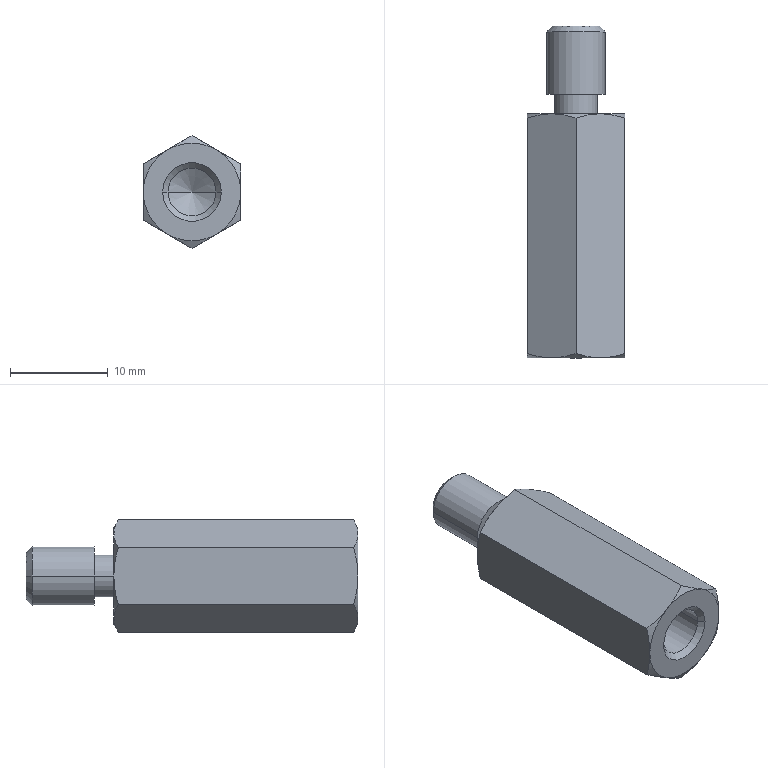Component | SolidWorks | RBE12-S10-L25-M6-N6.stp-1 | 1 solid | 34 faces | volume 2091 mm3 | cone 18 | plane 10 | cylinder 6 | commonest cylinder face diameters 6 x2 4.4 x2 4.917 x2